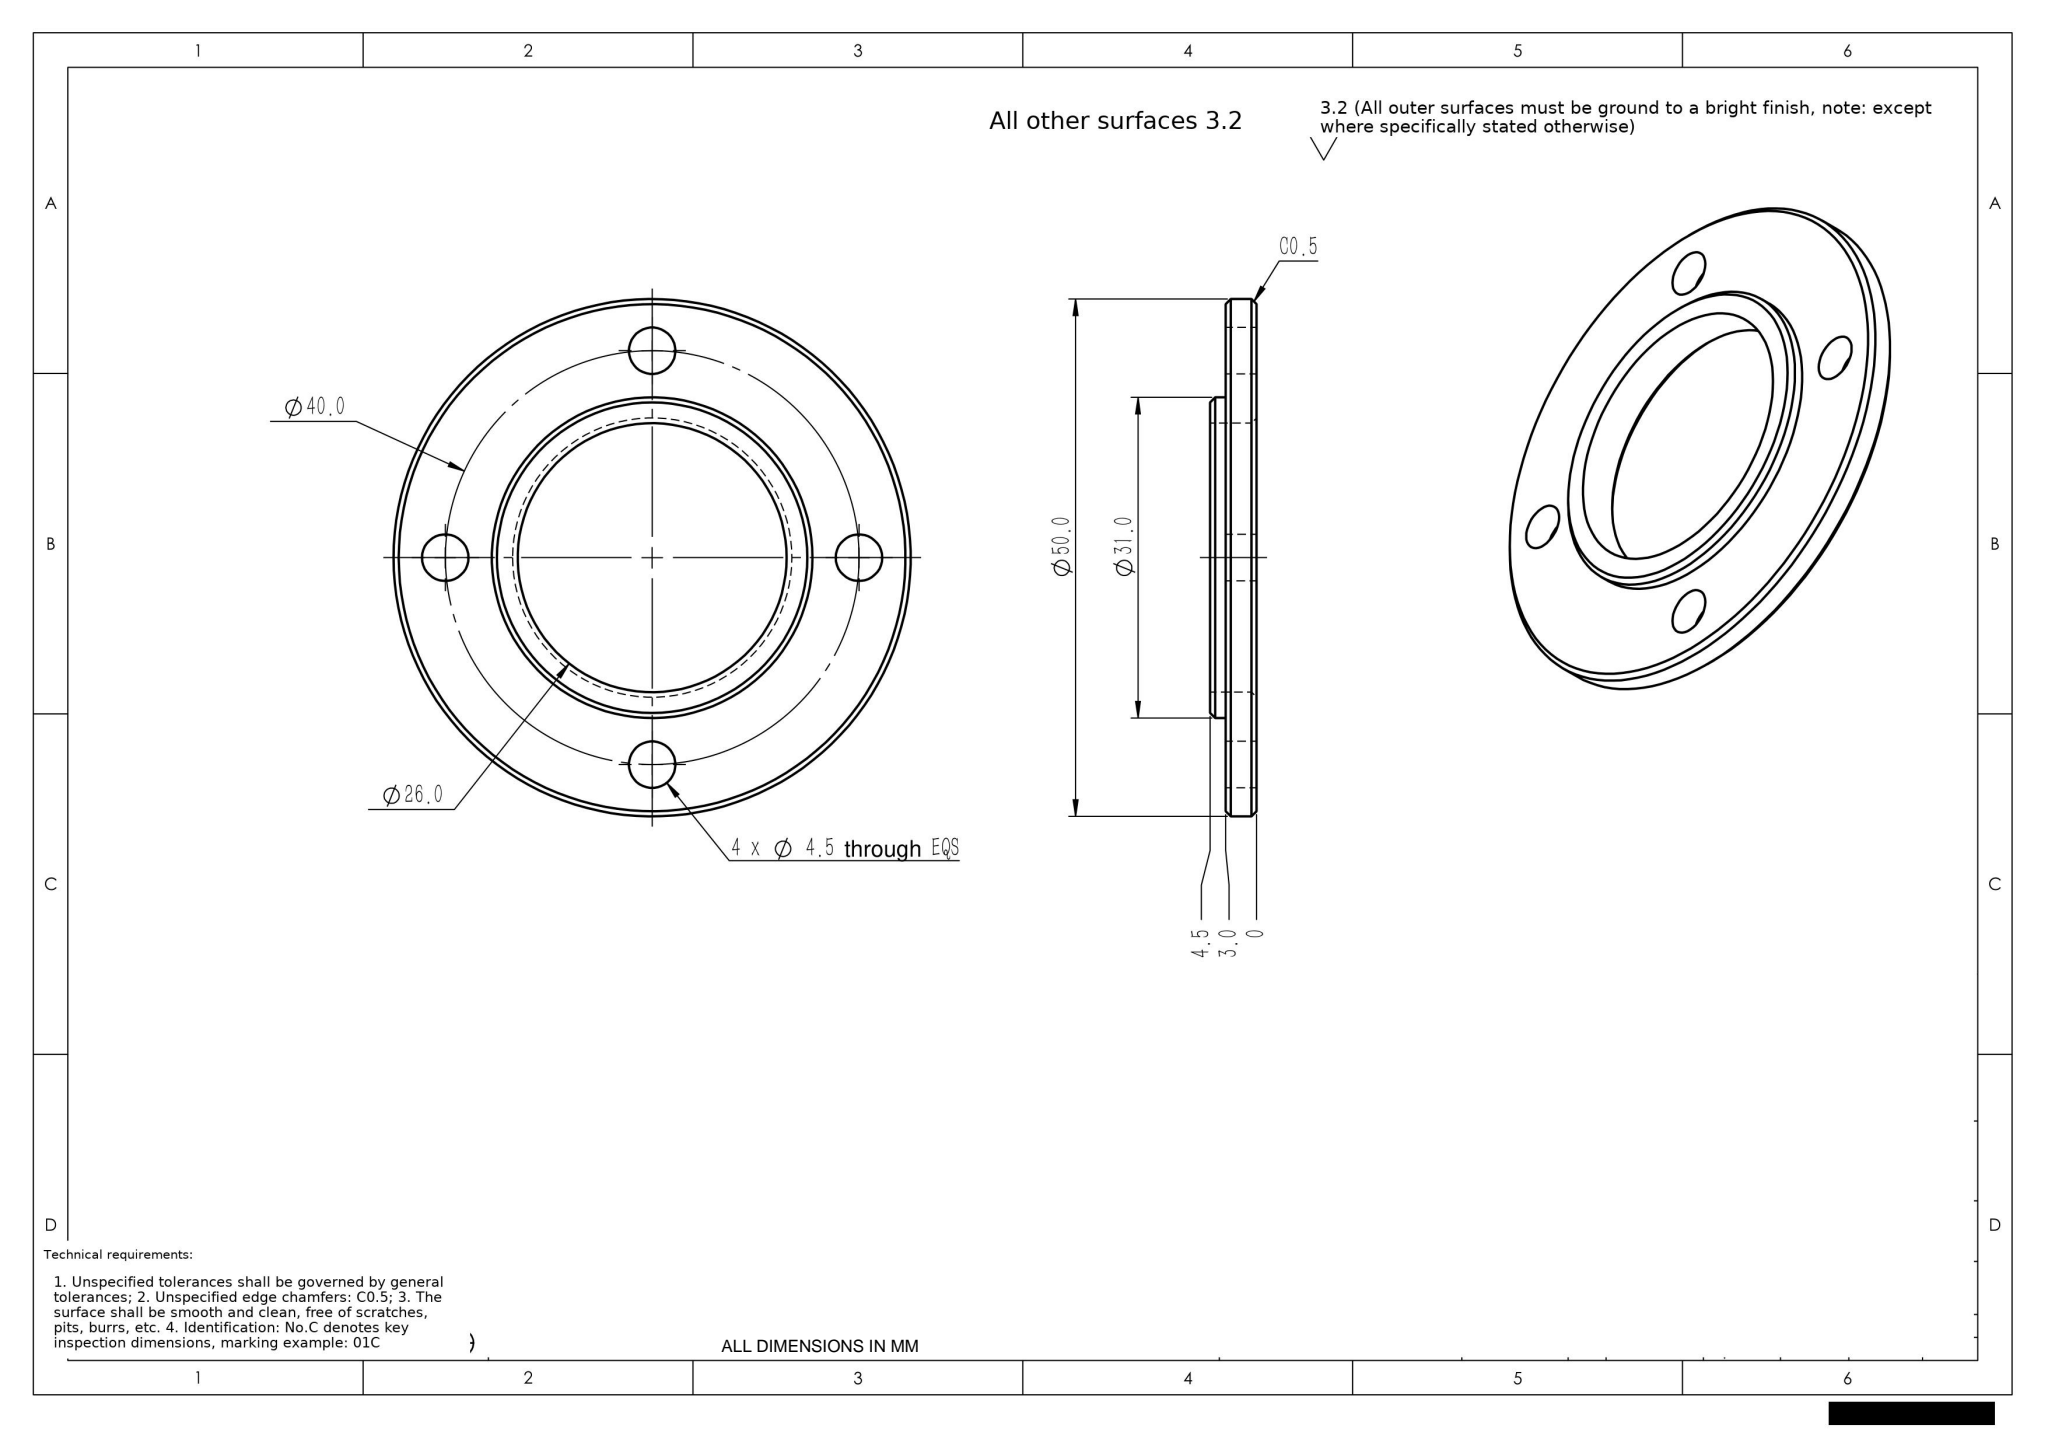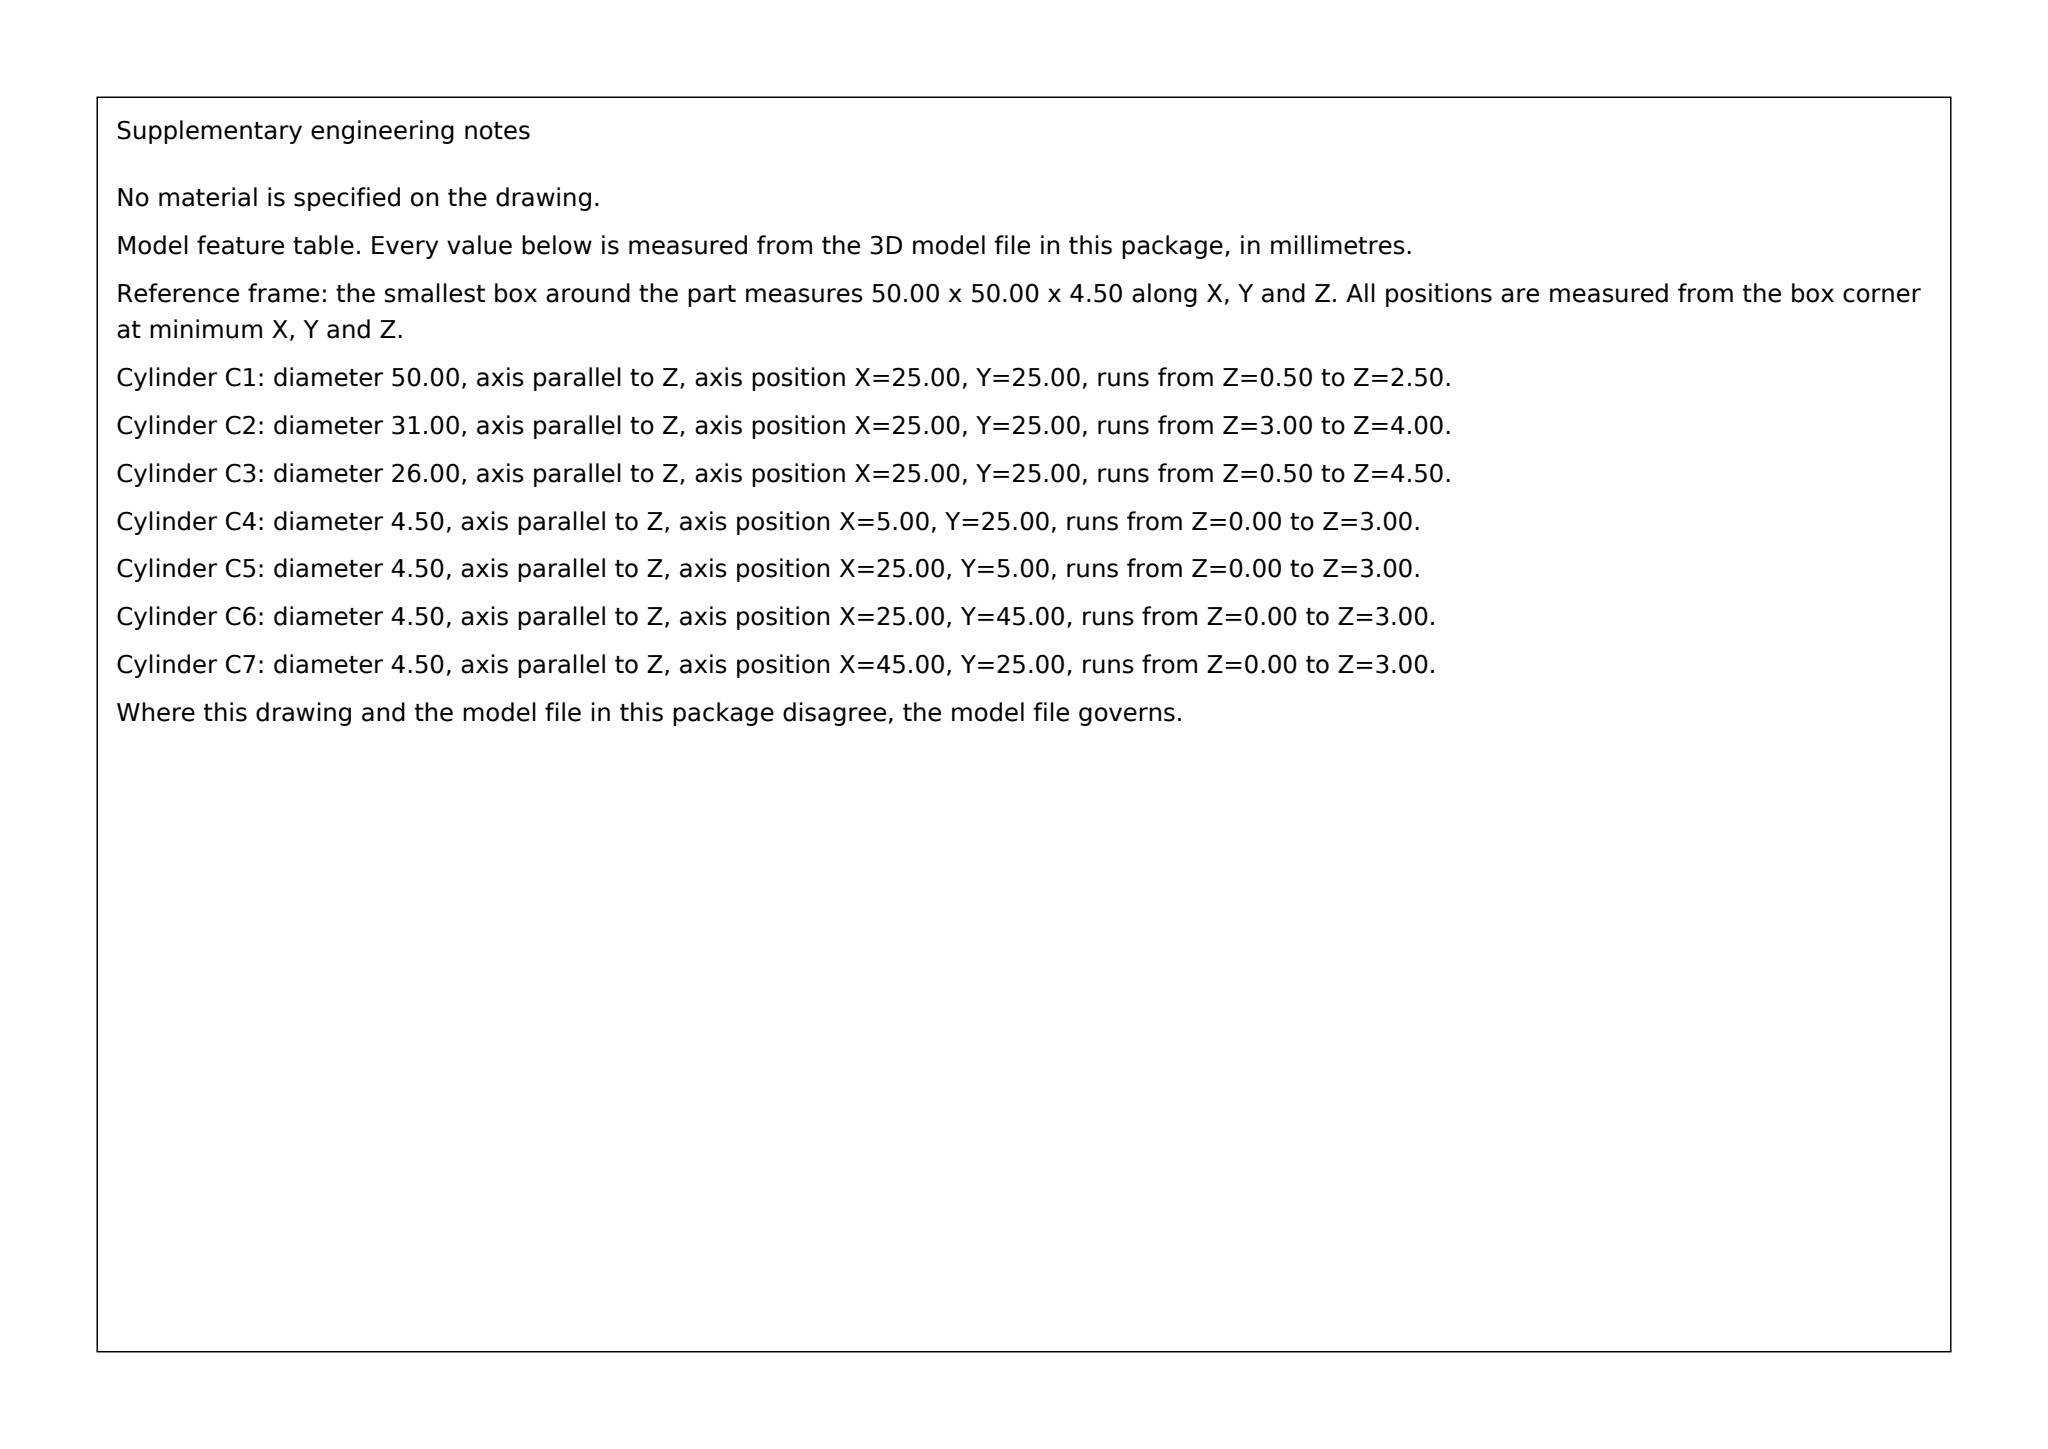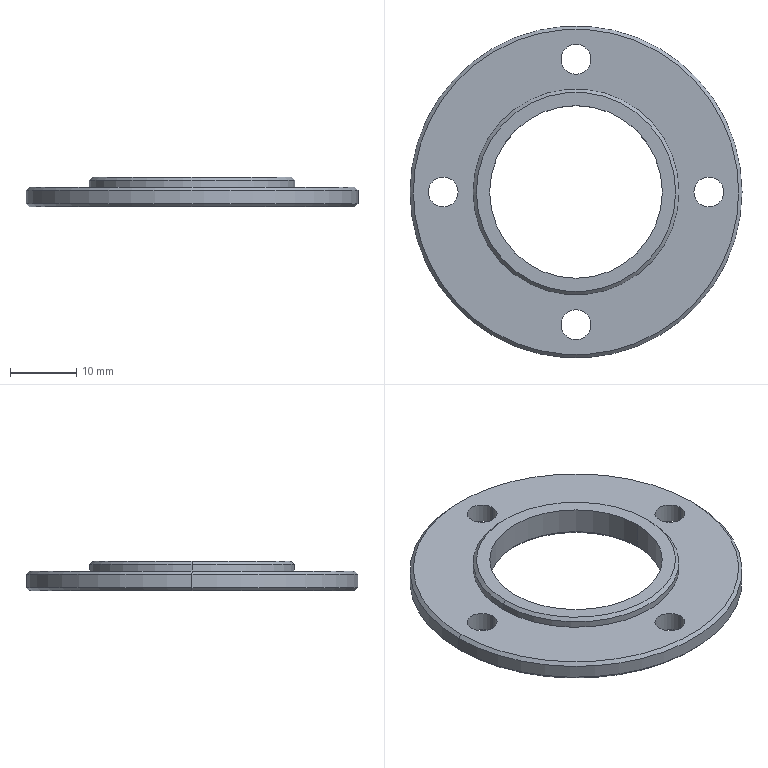Part | SolidWorks | mm | 1 solid | 25 faces | box 50 x 50 x 4.5 mm | volume 4381 mm3 | cylinder 14 | cone 8 | plane 3 | commonest cylinder face diameters 4.5 x8 26 x2 50 x2 31 x2
build123d program:
from build123d import *

# Parameters (mm, degrees)
SKETCH1_R                  = 15.5
BOSS_EXTRUDE1_DEPTH        = 1.5
SKETCH2_R                  = 25
BOSS_EXTRUDE2_DEPTH        = 3
SKETCH3_R                  = 13
CUT_EXTRUDE1_DEPTH         = 36.641
F_4_5_4_5_DIAMETER_HOLE1_D = 4.5
CHAMFER1_SIZE              = 0.5


with BuildPart() as part:
    # Sketch1 → Boss-Extrude1 (new body)
    with BuildSketch(Plane.XY):
        Circle(SKETCH1_R)
    extrude(amount=BOSS_EXTRUDE1_DEPTH)

    # Sketch2 → Boss-Extrude2 (add)
    with BuildSketch(Plane(origin=(0, 0, 0), x_dir=(-1, 0, 0), z_dir=(0, 0, -1))):
        Circle(SKETCH2_R)
    extrude(amount=BOSS_EXTRUDE2_DEPTH)

    # Sketch3 → Cut-Extrude1 (cut, through all)
    with BuildSketch(Plane.XY.offset(1.5)):
        Circle(SKETCH3_R)
    extrude(amount=-CUT_EXTRUDE1_DEPTH, mode=Mode.SUBTRACT)

    # 4.5 _4.5_ Diameter Hole1 (through all)
    with Locations(Plane(origin=(0, 0, -3), x_dir=(-1, 0, 0), z_dir=(0, 0, -1))):
        with Locations((0, -20), (0, 20), (-20, 0), (20, 0)):
            Hole(F_4_5_4_5_DIAMETER_HOLE1_D / 2)

    # Chamfer1
    chamfer1_edges = [part.edges().sort_by_distance(p)[0] for p in [
        (-13, 0, -3),
        (-15.5, 0, 1.5),
        (25, 0, 0),
        (25, 0, -3),
    ]]
    chamfer(chamfer1_edges, length=CHAMFER1_SIZE)


solid = part.part
STEP:
#1=CARTESIAN_POINT('',(15.,0.,1.5));
#2=VERTEX_POINT('',#1);
#3=CARTESIAN_POINT('',(-15.,0.,1.5));
#4=VERTEX_POINT('',#3);
#5=CARTESIAN_POINT('',(0.,0.,1.5));
#6=DIRECTION('',(0.,0.,1.));
#7=DIRECTION('',(1.,0.,0.));
#8=AXIS2_PLACEMENT_3D('',#5,#6,#7);
#9=CIRCLE('',#8,15.);
#10=EDGE_CURVE('',#2,#4,#9,.T.);
#11=ORIENTED_EDGE('',*,*,#10,.F.);
#12=CARTESIAN_POINT('',(15.5,0.,1.));
#13=VERTEX_POINT('',#12);
#14=CARTESIAN_POINT('',(15.,0.,1.5));
#15=DIRECTION('',(0.7071,0.,-0.7071));
#16=VECTOR('',#15,1000.);
#17=LINE('',#14,#16);
#18=EDGE_CURVE('',#2,#13,#17,.T.);
#19=ORIENTED_EDGE('',*,*,#18,.T.);
#20=CARTESIAN_POINT('',(-15.5,0.,1.));
#21=VERTEX_POINT('',#20);
#22=CARTESIAN_POINT('',(0.,0.,1.));
#23=DIRECTION('',(0.,0.,-1.));
#24=DIRECTION('',(1.,0.,0.));
#25=AXIS2_PLACEMENT_3D('',#22,#23,#24);
#26=CIRCLE('',#25,15.5);
#27=EDGE_CURVE('',#21,#13,#26,.T.);
#28=ORIENTED_EDGE('',*,*,#27,.F.);
#29=CARTESIAN_POINT('',(-15.,0.,1.5));
#30=DIRECTION('',(-0.7071,0.,-0.7071));
#31=VECTOR('',#30,1000.);
#32=LINE('',#29,#31);
#33=EDGE_CURVE('',#4,#21,#32,.T.);
#34=ORIENTED_EDGE('',*,*,#33,.F.);
#35=EDGE_LOOP('',(#11,#19,#28,#34));
#36=FACE_OUTER_BOUND('',#35,.T.);
#37=CARTESIAN_POINT('',(0.,0.,1.5));
#38=DIRECTION('',(0.,0.,-1.));
#39=DIRECTION('',(-1.,0.,0.));
#40=AXIS2_PLACEMENT_3D('',#37,#38,#39);
#41=CONICAL_SURFACE('',#40,15.,0.7854);
#42=ADVANCED_FACE('',(#36),#41,.T.);
#43=CARTESIAN_POINT('',(24.5,0.,0.));
#44=VERTEX_POINT('',#43);
#45=CARTESIAN_POINT('',(-24.5,0.,0.));
#46=VERTEX_POINT('',#45);
#47=CARTESIAN_POINT('',(0.,0.,0.));
#48=DIRECTION('',(0.,0.,1.));
#49=DIRECTION('',(-1.,0.,0.));
#50=AXIS2_PLACEMENT_3D('',#47,#48,#49);
#51=CIRCLE('',#50,24.5);
#52=EDGE_CURVE('',#44,#46,#51,.T.);
#53=ORIENTED_EDGE('',*,*,#52,.F.);
#54=CARTESIAN_POINT('',(25.,0.,-0.5));
#55=VERTEX_POINT('',#54);
#56=CARTESIAN_POINT('',(25.,0.,-0.5));
#57=DIRECTION('',(0.7071,0.,-0.7071));
#58=VECTOR('',#57,1000.);
#59=LINE('',#56,#58);
#60=EDGE_CURVE('',#44,#55,#59,.T.);
#61=ORIENTED_EDGE('',*,*,#60,.T.);
#62=CARTESIAN_POINT('',(-25.,0.,-0.5));
#63=VERTEX_POINT('',#62);
#64=CARTESIAN_POINT('',(0.,0.,-0.5));
#65=DIRECTION('',(0.,0.,-1.));
#66=DIRECTION('',(-1.,0.,0.));
#67=AXIS2_PLACEMENT_3D('',#64,#65,#66);
#68=CIRCLE('',#67,25.);
#69=EDGE_CURVE('',#63,#55,#68,.T.);
#70=ORIENTED_EDGE('',*,*,#69,.F.);
#71=CARTESIAN_POINT('',(-25.,0.,-0.5));
#72=DIRECTION('',(-0.7071,0.,-0.7071));
#73=VECTOR('',#72,1000.);
#74=LINE('',#71,#73);
#75=EDGE_CURVE('',#46,#63,#74,.T.);
#76=ORIENTED_EDGE('',*,*,#75,.F.);
#77=EDGE_LOOP('',(#53,#61,#70,#76));
#78=FACE_OUTER_BOUND('',#77,.T.);
#79=CARTESIAN_POINT('',(0.,0.,-0.5));
#80=DIRECTION('',(0.,0.,-1.));
#81=DIRECTION('',(-1.,0.,0.));
#82=AXIS2_PLACEMENT_3D('',#79,#80,#81);
#83=CONICAL_SURFACE('',#82,25.,0.7854);
#84=ADVANCED_FACE('',(#78),#83,.T.);
#85=CARTESIAN_POINT('',(-24.5,0.,-3.));
#86=VERTEX_POINT('',#85);
#87=CARTESIAN_POINT('',(24.5,0.,-3.));
#88=VERTEX_POINT('',#87);
#89=CARTESIAN_POINT('',(0.,0.,-3.));
#90=DIRECTION('',(0.,0.,-1.));
#91=DIRECTION('',(-1.,0.,0.));
#92=AXIS2_PLACEMENT_3D('',#89,#90,#91);
#93=CIRCLE('',#92,24.5);
#94=EDGE_CURVE('',#86,#88,#93,.T.);
#95=ORIENTED_EDGE('',*,*,#94,.F.);
#96=CARTESIAN_POINT('',(-25.,0.,-2.5));
#97=VERTEX_POINT('',#96);
#98=CARTESIAN_POINT('',(-24.5,0.,-3.));
#99=DIRECTION('',(-0.7071,0.,0.7071));
#100=VECTOR('',#99,1000.);
#101=LINE('',#98,#100);
#102=EDGE_CURVE('',#86,#97,#101,.T.);
#103=ORIENTED_EDGE('',*,*,#102,.T.);
#104=CARTESIAN_POINT('',(25.,0.,-2.5));
#105=VERTEX_POINT('',#104);
#106=CARTESIAN_POINT('',(0.,0.,-2.5));
#107=DIRECTION('',(0.,0.,1.));
#108=DIRECTION('',(-1.,0.,0.));
#109=AXIS2_PLACEMENT_3D('',#106,#107,#108);
#110=CIRCLE('',#109,25.);
#111=EDGE_CURVE('',#105,#97,#110,.T.);
#112=ORIENTED_EDGE('',*,*,#111,.F.);
#113=CARTESIAN_POINT('',(24.5,0.,-3.));
#114=DIRECTION('',(0.7071,0.,0.7071));
#115=VECTOR('',#114,1000.);
#116=LINE('',#113,#115);
#117=EDGE_CURVE('',#88,#105,#116,.T.);
#118=ORIENTED_EDGE('',*,*,#117,.F.);
#119=EDGE_LOOP('',(#95,#103,#112,#118));
#120=FACE_OUTER_BOUND('',#119,.T.);
#121=CARTESIAN_POINT('',(0.,0.,-3.));
#122=DIRECTION('',(0.,0.,1.));
#123=DIRECTION('',(1.,0.,0.));
#124=AXIS2_PLACEMENT_3D('',#121,#122,#123);
#125=CONICAL_SURFACE('',#124,24.5,0.7854);
#126=ADVANCED_FACE('',(#120),#125,.T.);
#127=CARTESIAN_POINT('',(13.,0.,-2.5));
#128=VERTEX_POINT('',#127);
#129=CARTESIAN_POINT('',(-13.,0.,-2.5));
#130=VERTEX_POINT('',#129);
#131=CARTESIAN_POINT('',(0.,0.,-2.5));
#132=DIRECTION('',(0.,0.,-1.));
#133=DIRECTION('',(-1.,0.,0.));
#134=AXIS2_PLACEMENT_3D('',#131,#132,#133);
#135=CIRCLE('',#134,13.);
#136=EDGE_CURVE('',#128,#130,#135,.T.);
#137=ORIENTED_EDGE('',*,*,#136,.F.);
#138=CARTESIAN_POINT('',(13.5,0.,-3.));
#139=VERTEX_POINT('',#138);
#140=CARTESIAN_POINT('',(13.5,0.,-3.));
#141=DIRECTION('',(0.7071,0.,-0.7071));
#142=VECTOR('',#141,1000.);
#143=LINE('',#140,#142);
#144=EDGE_CURVE('',#128,#139,#143,.T.);
#145=ORIENTED_EDGE('',*,*,#144,.T.);
#146=CARTESIAN_POINT('',(-13.5,0.,-3.));
#147=VERTEX_POINT('',#146);
#148=CARTESIAN_POINT('',(0.,0.,-3.));
#149=DIRECTION('',(0.,0.,1.));
#150=DIRECTION('',(-1.,0.,0.));
#151=AXIS2_PLACEMENT_3D('',#148,#149,#150);
#152=CIRCLE('',#151,13.5);
#153=EDGE_CURVE('',#147,#139,#152,.T.);
#154=ORIENTED_EDGE('',*,*,#153,.F.);
#155=CARTESIAN_POINT('',(-13.5,0.,-3.));
#156=DIRECTION('',(-0.7071,0.,-0.7071));
#157=VECTOR('',#156,1000.);
#158=LINE('',#155,#157);
#159=EDGE_CURVE('',#130,#147,#158,.T.);
#160=ORIENTED_EDGE('',*,*,#159,.F.);
#161=EDGE_LOOP('',(#137,#145,#154,#160));
#162=FACE_OUTER_BOUND('',#161,.T.);
#163=CARTESIAN_POINT('',(0.,0.,-3.));
#164=DIRECTION('',(0.,0.,-1.));
#165=DIRECTION('',(-1.,0.,0.));
#166=AXIS2_PLACEMENT_3D('',#163,#164,#165);
#167=CONICAL_SURFACE('',#166,13.5,0.7854);
#168=ADVANCED_FACE('',(#162),#167,.F.);
#169=CARTESIAN_POINT('',(2.25,-20.,0.));
#170=VERTEX_POINT('',#169);
#171=CARTESIAN_POINT('',(-2.25,-20.,0.));
#172=VERTEX_POINT('',#171);
#173=CARTESIAN_POINT('',(0.,-20.,0.));
#174=DIRECTION('',(0.,0.,-1.));
#175=DIRECTION('',(-1.,0.,0.));
#176=AXIS2_PLACEMENT_3D('',#173,#174,#175);
#177=CIRCLE('',#176,2.25);
#178=EDGE_CURVE('',#170,#172,#177,.T.);
#179=ORIENTED_EDGE('',*,*,#178,.F.);
#180=CARTESIAN_POINT('',(2.25,-20.,-3.));
#181=VERTEX_POINT('',#180);
#182=CARTESIAN_POINT('',(2.25,-20.,-3.));
#183=DIRECTION('',(0.,0.,-1.));
#184=VECTOR('',#183,1000.);
#185=LINE('',#182,#184);
#186=EDGE_CURVE('',#170,#181,#185,.T.);
#187=ORIENTED_EDGE('',*,*,#186,.T.);
#188=CARTESIAN_POINT('',(-2.25,-20.,-3.));
#189=VERTEX_POINT('',#188);
#190=CARTESIAN_POINT('',(0.,-20.,-3.));
#191=DIRECTION('',(0.,0.,-1.));
#192=DIRECTION('',(-1.,0.,0.));
#193=AXIS2_PLACEMENT_3D('',#190,#191,#192);
#194=CIRCLE('',#193,2.25);
#195=EDGE_CURVE('',#181,#189,#194,.T.);
#196=ORIENTED_EDGE('',*,*,#195,.T.);
#197=CARTESIAN_POINT('',(-2.25,-20.,-3.));
#198=DIRECTION('',(0.,0.,-1.));
#199=VECTOR('',#198,1000.);
#200=LINE('',#197,#199);
#201=EDGE_CURVE('',#172,#189,#200,.T.);
#202=ORIENTED_EDGE('',*,*,#201,.F.);
#203=EDGE_LOOP('',(#179,#187,#196,#202));
#204=FACE_OUTER_BOUND('',#203,.T.);
#205=CARTESIAN_POINT('',(0.,-20.,-3.));
#206=DIRECTION('',(0.,0.,-1.));
#207=DIRECTION('',(-1.,0.,0.));
#208=AXIS2_PLACEMENT_3D('',#205,#206,#207);
#209=CYLINDRICAL_SURFACE('',#208,2.25);
#210=ADVANCED_FACE('',(#204),#209,.F.);
#211=CARTESIAN_POINT('',(2.25,20.,0.));
#212=VERTEX_POINT('',#211);
#213=CARTESIAN_POINT('',(-2.25,20.,0.));
#214=VERTEX_POINT('',#213);
#215=CARTESIAN_POINT('',(0.,20.,0.));
#216=DIRECTION('',(0.,0.,-1.));
#217=DIRECTION('',(-1.,0.,0.));
#218=AXIS2_PLACEMENT_3D('',#215,#216,#217);
#219=CIRCLE('',#218,2.25);
#220=EDGE_CURVE('',#212,#214,#219,.T.);
#221=ORIENTED_EDGE('',*,*,#220,.F.);
#222=CARTESIAN_POINT('',(2.25,20.,-3.));
#223=VERTEX_POINT('',#222);
#224=CARTESIAN_POINT('',(2.25,20.,-3.));
#225=DIRECTION('',(0.,0.,-1.));
#226=VECTOR('',#225,1000.);
#227=LINE('',#224,#226);
#228=EDGE_CURVE('',#212,#223,#227,.T.);
#229=ORIENTED_EDGE('',*,*,#228,.T.);
#230=CARTESIAN_POINT('',(-2.25,20.,-3.));
#231=VERTEX_POINT('',#230);
#232=CARTESIAN_POINT('',(0.,20.,-3.));
#233=DIRECTION('',(0.,0.,-1.));
#234=DIRECTION('',(-1.,0.,0.));
#235=AXIS2_PLACEMENT_3D('',#232,#233,#234);
#236=CIRCLE('',#235,2.25);
#237=EDGE_CURVE('',#223,#231,#236,.T.);
#238=ORIENTED_EDGE('',*,*,#237,.T.);
#239=CARTESIAN_POINT('',(-2.25,20.,-3.));
#240=DIRECTION('',(0.,0.,-1.));
#241=VECTOR('',#240,1000.);
#242=LINE('',#239,#241);
#243=EDGE_CURVE('',#214,#231,#242,.T.);
#244=ORIENTED_EDGE('',*,*,#243,.F.);
#245=EDGE_LOOP('',(#221,#229,#238,#244));
#246=FACE_OUTER_BOUND('',#245,.T.);
#247=CARTESIAN_POINT('',(0.,20.,-3.));
#248=DIRECTION('',(0.,0.,-1.));
#249=DIRECTION('',(-1.,0.,0.));
#250=AXIS2_PLACEMENT_3D('',#247,#248,#249);
#251=CYLINDRICAL_SURFACE('',#250,2.25);
#252=ADVANCED_FACE('',(#246),#251,.F.);
#253=CARTESIAN_POINT('',(22.25,0.,0.));
#254=VERTEX_POINT('',#253);
#255=CARTESIAN_POINT('',(17.75,0.,0.));
#256=VERTEX_POINT('',#255);
#257=CARTESIAN_POINT('',(20.,0.,0.));
#258=DIRECTION('',(0.,0.,-1.));
#259=DIRECTION('',(-1.,0.,0.));
#260=AXIS2_PLACEMENT_3D('',#257,#258,#259);
#261=CIRCLE('',#260,2.25);
#262=EDGE_CURVE('',#254,#256,#261,.T.);
#263=ORIENTED_EDGE('',*,*,#262,.F.);
#264=CARTESIAN_POINT('',(22.25,0.,-3.));
#265=VERTEX_POINT('',#264);
#266=CARTESIAN_POINT('',(22.25,0.,-3.));
#267=DIRECTION('',(0.,0.,-1.));
#268=VECTOR('',#267,1000.);
#269=LINE('',#266,#268);
#270=EDGE_CURVE('',#254,#265,#269,.T.);
#271=ORIENTED_EDGE('',*,*,#270,.T.);
#272=CARTESIAN_POINT('',(17.75,0.,-3.));
#273=VERTEX_POINT('',#272);
#274=CARTESIAN_POINT('',(20.,0.,-3.));
#275=DIRECTION('',(0.,0.,-1.));
#276=DIRECTION('',(-1.,0.,0.));
#277=AXIS2_PLACEMENT_3D('',#274,#275,#276);
#278=CIRCLE('',#277,2.25);
#279=EDGE_CURVE('',#265,#273,#278,.T.);
#280=ORIENTED_EDGE('',*,*,#279,.T.);
#281=CARTESIAN_POINT('',(17.75,0.,-3.));
#282=DIRECTION('',(0.,0.,-1.));
#283=VECTOR('',#282,1000.);
#284=LINE('',#281,#283);
#285=EDGE_CURVE('',#256,#273,#284,.T.);
#286=ORIENTED_EDGE('',*,*,#285,.F.);
#287=EDGE_LOOP('',(#263,#271,#280,#286));
#288=FACE_OUTER_BOUND('',#287,.T.);
#289=CARTESIAN_POINT('',(20.,0.,-3.));
#290=DIRECTION('',(0.,0.,-1.));
#291=DIRECTION('',(-1.,0.,0.));
#292=AXIS2_PLACEMENT_3D('',#289,#290,#291);
#293=CYLINDRICAL_SURFACE('',#292,2.25);
#294=ADVANCED_FACE('',(#288),#293,.F.);
#295=CARTESIAN_POINT('',(-17.75,0.,0.));
#296=VERTEX_POINT('',#295);
#297=CARTESIAN_POINT('',(-22.25,0.,0.));
#298=VERTEX_POINT('',#297);
#299=CARTESIAN_POINT('',(-20.,0.,0.));
#300=DIRECTION('',(0.,0.,-1.));
#301=DIRECTION('',(-1.,0.,0.));
#302=AXIS2_PLACEMENT_3D('',#299,#300,#301);
#303=CIRCLE('',#302,2.25);
#304=EDGE_CURVE('',#296,#298,#303,.T.);
#305=ORIENTED_EDGE('',*,*,#304,.F.);
#306=CARTESIAN_POINT('',(-17.75,0.,-3.));
#307=VERTEX_POINT('',#306);
#308=CARTESIAN_POINT('',(-17.75,0.,-3.));
#309=DIRECTION('',(0.,0.,-1.));
#310=VECTOR('',#309,1000.);
#311=LINE('',#308,#310);
#312=EDGE_CURVE('',#296,#307,#311,.T.);
#313=ORIENTED_EDGE('',*,*,#312,.T.);
#314=CARTESIAN_POINT('',(-22.25,0.,-3.));
#315=VERTEX_POINT('',#314);
#316=CARTESIAN_POINT('',(-20.,0.,-3.));
#317=DIRECTION('',(0.,0.,-1.));
#318=DIRECTION('',(-1.,0.,0.));
#319=AXIS2_PLACEMENT_3D('',#316,#317,#318);
#320=CIRCLE('',#319,2.25);
#321=EDGE_CURVE('',#307,#315,#320,.T.);
#322=ORIENTED_EDGE('',*,*,#321,.T.);
#323=CARTESIAN_POINT('',(-22.25,0.,-3.));
#324=DIRECTION('',(0.,0.,-1.));
#325=VECTOR('',#324,1000.);
#326=LINE('',#323,#325);
#327=EDGE_CURVE('',#298,#315,#326,.T.);
#328=ORIENTED_EDGE('',*,*,#327,.F.);
#329=EDGE_LOOP('',(#305,#313,#322,#328));
#330=FACE_OUTER_BOUND('',#329,.T.);
#331=CARTESIAN_POINT('',(-20.,0.,-3.));
#332=DIRECTION('',(0.,0.,-1.));
#333=DIRECTION('',(-1.,0.,0.));
#334=AXIS2_PLACEMENT_3D('',#331,#332,#333);
#335=CYLINDRICAL_SURFACE('',#334,2.25);
#336=ADVANCED_FACE('',(#330),#335,.F.);
#337=ORIENTED_EDGE('',*,*,#136,.T.);
#338=CARTESIAN_POINT('',(-13.,0.,1.5));
#339=VERTEX_POINT('',#338);
#340=CARTESIAN_POINT('',(-13.,0.,-3.));
#341=DIRECTION('',(0.,0.,1.));
#342=VECTOR('',#341,1000.);
#343=LINE('',#340,#342);
#344=EDGE_CURVE('',#130,#339,#343,.T.);
#345=ORIENTED_EDGE('',*,*,#344,.T.);
#346=CARTESIAN_POINT('',(13.,0.,1.5));
#347=VERTEX_POINT('',#346);
#348=CARTESIAN_POINT('',(0.,0.,1.5));
#349=DIRECTION('',(0.,0.,1.));
#350=DIRECTION('',(1.,0.,0.));
#351=AXIS2_PLACEMENT_3D('',#348,#349,#350);
#352=CIRCLE('',#351,13.);
#353=EDGE_CURVE('',#339,#347,#352,.T.);
#354=ORIENTED_EDGE('',*,*,#353,.T.);
#355=CARTESIAN_POINT('',(13.,0.,-3.));
#356=DIRECTION('',(0.,0.,1.));
#357=VECTOR('',#356,1000.);
#358=LINE('',#355,#357);
#359=EDGE_CURVE('',#128,#347,#358,.T.);
#360=ORIENTED_EDGE('',*,*,#359,.F.);
#361=EDGE_LOOP('',(#337,#345,#354,#360));
#362=FACE_OUTER_BOUND('',#361,.T.);
#363=CARTESIAN_POINT('',(0.,0.,-3.));
#364=DIRECTION('',(0.,0.,1.));
#365=DIRECTION('',(1.,0.,0.));
#366=AXIS2_PLACEMENT_3D('',#363,#364,#365);
#367=CYLINDRICAL_SURFACE('',#366,13.);
#368=ADVANCED_FACE('',(#362),#367,.F.);
#369=ORIENTED_EDGE('',*,*,#111,.T.);
#370=CARTESIAN_POINT('',(-25.,0.,-3.));
#371=DIRECTION('',(0.,0.,1.));
#372=VECTOR('',#371,1000.);
#373=LINE('',#370,#372);
#374=EDGE_CURVE('',#97,#63,#373,.T.);
#375=ORIENTED_EDGE('',*,*,#374,.T.);
#376=ORIENTED_EDGE('',*,*,#69,.T.);
#377=CARTESIAN_POINT('',(25.,0.,-3.));
#378=DIRECTION('',(0.,0.,1.));
#379=VECTOR('',#378,1000.);
#380=LINE('',#377,#379);
#381=EDGE_CURVE('',#105,#55,#380,.T.);
#382=ORIENTED_EDGE('',*,*,#381,.F.);
#383=EDGE_LOOP('',(#369,#375,#376,#382));
#384=FACE_OUTER_BOUND('',#383,.T.);
#385=CARTESIAN_POINT('',(0.,0.,-3.));
#386=DIRECTION('',(0.,0.,1.));
#387=DIRECTION('',(1.,0.,0.));
#388=AXIS2_PLACEMENT_3D('',#385,#386,#387);
#389=CYLINDRICAL_SURFACE('',#388,25.);
#390=ADVANCED_FACE('',(#384),#389,.T.);
#391=ORIENTED_EDGE('',*,*,#27,.T.);
#392=CARTESIAN_POINT('',(15.5,0.,0.));
#393=VERTEX_POINT('',#392);
#394=CARTESIAN_POINT('',(15.5,0.,1.5));
#395=DIRECTION('',(0.,0.,-1.));
#396=VECTOR('',#395,1000.);
#397=LINE('',#394,#396);
#398=EDGE_CURVE('',#13,#393,#397,.T.);
#399=ORIENTED_EDGE('',*,*,#398,.T.);
#400=CARTESIAN_POINT('',(-15.5,0.,0.));
#401=VERTEX_POINT('',#400);
#402=CARTESIAN_POINT('',(0.,0.,0.));
#403=DIRECTION('',(0.,0.,-1.));
#404=DIRECTION('',(-1.,0.,0.));
#405=AXIS2_PLACEMENT_3D('',#402,#403,#404);
#406=CIRCLE('',#405,15.5);
#407=EDGE_CURVE('',#401,#393,#406,.T.);
#408=ORIENTED_EDGE('',*,*,#407,.F.);
#409=CARTESIAN_POINT('',(-15.5,0.,1.5));
#410=DIRECTION('',(0.,0.,-1.));
#411=VECTOR('',#410,1000.);
#412=LINE('',#409,#411);
#413=EDGE_CURVE('',#21,#401,#412,.T.);
#414=ORIENTED_EDGE('',*,*,#413,.F.);
#415=EDGE_LOOP('',(#391,#399,#408,#414));
#416=FACE_OUTER_BOUND('',#415,.T.);
#417=CARTESIAN_POINT('',(0.,0.,1.5));
#418=DIRECTION('',(0.,0.,-1.));
#419=DIRECTION('',(-1.,0.,0.));
#420=AXIS2_PLACEMENT_3D('',#417,#418,#419);
#421=CYLINDRICAL_SURFACE('',#420,15.5);
#422=ADVANCED_FACE('',(#416),#421,.T.);
#423=ORIENTED_EDGE('',*,*,#398,.F.);
#424=CARTESIAN_POINT('',(0.,0.,1.));
#425=DIRECTION('',(0.,0.,-1.));
#426=DIRECTION('',(1.,0.,0.));
#427=AXIS2_PLACEMENT_3D('',#424,#425,#426);
#428=CIRCLE('',#427,15.5);
#429=EDGE_CURVE('',#13,#21,#428,.T.);
#430=ORIENTED_EDGE('',*,*,#429,.T.);
#431=ORIENTED_EDGE('',*,*,#413,.T.);
#432=CARTESIAN_POINT('',(0.,0.,0.));
#433=DIRECTION('',(0.,0.,-1.));
#434=DIRECTION('',(-1.,0.,0.));
#435=AXIS2_PLACEMENT_3D('',#432,#433,#434);
#436=CIRCLE('',#435,15.5);
#437=EDGE_CURVE('',#393,#401,#436,.T.);
#438=ORIENTED_EDGE('',*,*,#437,.F.);
#439=EDGE_LOOP('',(#423,#430,#431,#438));
#440=FACE_OUTER_BOUND('',#439,.T.);
#441=CARTESIAN_POINT('',(0.,0.,1.5));
#442=DIRECTION('',(0.,0.,-1.));
#443=DIRECTION('',(-1.,0.,0.));
#444=AXIS2_PLACEMENT_3D('',#441,#442,#443);
#445=CYLINDRICAL_SURFACE('',#444,15.5);
#446=ADVANCED_FACE('',(#440),#445,.T.);
#447=CARTESIAN_POINT('',(0.,0.,1.5));
#448=DIRECTION('',(0.,0.,1.));
#449=DIRECTION('',(1.,0.,0.));
#450=AXIS2_PLACEMENT_3D('',#447,#448,#449);
#451=CIRCLE('',#450,15.);
#452=EDGE_CURVE('',#4,#2,#451,.T.);
#453=ORIENTED_EDGE('',*,*,#452,.T.);
#454=ORIENTED_EDGE('',*,*,#10,.T.);
#455=EDGE_LOOP('',(#453,#454));
#456=FACE_OUTER_BOUND('',#455,.T.);
#457=CARTESIAN_POINT('',(0.,0.,1.5));
#458=DIRECTION('',(0.,0.,1.));
#459=DIRECTION('',(1.,0.,0.));
#460=AXIS2_PLACEMENT_3D('',#457,#458,#459);
#461=CIRCLE('',#460,13.);
#462=EDGE_CURVE('',#347,#339,#461,.T.);
#463=ORIENTED_EDGE('',*,*,#462,.F.);
#464=ORIENTED_EDGE('',*,*,#353,.F.);
#465=EDGE_LOOP('',(#463,#464));
#466=FACE_BOUND('',#465,.T.);
#467=CARTESIAN_POINT('',(0.,0.,1.5));
#468=DIRECTION('',(0.,0.,1.));
#469=DIRECTION('',(1.,0.,0.));
#470=AXIS2_PLACEMENT_3D('',#467,#468,#469);
#471=PLANE('',#470);
#472=ADVANCED_FACE('',(#456,#466),#471,.T.);
#473=ORIENTED_EDGE('',*,*,#374,.F.);
#474=CARTESIAN_POINT('',(0.,0.,-2.5));
#475=DIRECTION('',(0.,0.,1.));
#476=DIRECTION('',(-1.,0.,0.));
#477=AXIS2_PLACEMENT_3D('',#474,#475,#476);
#478=CIRCLE('',#477,25.);
#479=EDGE_CURVE('',#97,#105,#478,.T.);
#480=ORIENTED_EDGE('',*,*,#479,.T.);
#481=ORIENTED_EDGE('',*,*,#381,.T.);
#482=CARTESIAN_POINT('',(0.,0.,-0.5));
#483=DIRECTION('',(0.,0.,-1.));
#484=DIRECTION('',(-1.,0.,0.));
#485=AXIS2_PLACEMENT_3D('',#482,#483,#484);
#486=CIRCLE('',#485,25.);
#487=EDGE_CURVE('',#55,#63,#486,.T.);
#488=ORIENTED_EDGE('',*,*,#487,.T.);
#489=EDGE_LOOP('',(#473,#480,#481,#488));
#490=FACE_OUTER_BOUND('',#489,.T.);
#491=CARTESIAN_POINT('',(0.,0.,-3.));
#492=DIRECTION('',(0.,0.,1.));
#493=DIRECTION('',(1.,0.,0.));
#494=AXIS2_PLACEMENT_3D('',#491,#492,#493);
#495=CYLINDRICAL_SURFACE('',#494,25.);
#496=ADVANCED_FACE('',(#490),#495,.T.);
#497=ORIENTED_EDGE('',*,*,#153,.T.);
#498=CARTESIAN_POINT('',(0.,0.,-3.));
#499=DIRECTION('',(0.,0.,1.));
#500=DIRECTION('',(-1.,0.,0.));
#501=AXIS2_PLACEMENT_3D('',#498,#499,#500);
#502=CIRCLE('',#501,13.5);
#503=EDGE_CURVE('',#139,#147,#502,.T.);
#504=ORIENTED_EDGE('',*,*,#503,.T.);
#505=EDGE_LOOP('',(#497,#504));
#506=FACE_BOUND('',#505,.T.);
#507=CARTESIAN_POINT('',(0.,0.,-3.));
#508=DIRECTION('',(0.,0.,-1.));
#509=DIRECTION('',(-1.,0.,0.));
#510=AXIS2_PLACEMENT_3D('',#507,#508,#509);
#511=CIRCLE('',#510,24.5);
#512=EDGE_CURVE('',#88,#86,#511,.T.);
#513=ORIENTED_EDGE('',*,*,#512,.T.);
#514=ORIENTED_EDGE('',*,*,#94,.T.);
#515=EDGE_LOOP('',(#513,#514));
#516=FACE_OUTER_BOUND('',#515,.T.);
#517=CARTESIAN_POINT('',(0.,-20.,-3.));
#518=DIRECTION('',(0.,0.,-1.));
#519=DIRECTION('',(-1.,0.,0.));
#520=AXIS2_PLACEMENT_3D('',#517,#518,#519);
#521=CIRCLE('',#520,2.25);
#522=EDGE_CURVE('',#189,#181,#521,.T.);
#523=ORIENTED_EDGE('',*,*,#522,.F.);
#524=ORIENTED_EDGE('',*,*,#195,.F.);
#525=EDGE_LOOP('',(#523,#524));
#526=FACE_BOUND('',#525,.T.);
#527=CARTESIAN_POINT('',(0.,20.,-3.));
#528=DIRECTION('',(0.,0.,-1.));
#529=DIRECTION('',(-1.,0.,0.));
#530=AXIS2_PLACEMENT_3D('',#527,#528,#529);
#531=CIRCLE('',#530,2.25);
#532=EDGE_CURVE('',#231,#223,#531,.T.);
#533=ORIENTED_EDGE('',*,*,#532,.F.);
#534=ORIENTED_EDGE('',*,*,#237,.F.);
#535=EDGE_LOOP('',(#533,#534));
#536=FACE_BOUND('',#535,.T.);
#537=CARTESIAN_POINT('',(20.,0.,-3.));
#538=DIRECTION('',(0.,0.,-1.));
#539=DIRECTION('',(-1.,0.,0.));
#540=AXIS2_PLACEMENT_3D('',#537,#538,#539);
#541=CIRCLE('',#540,2.25);
#542=EDGE_CURVE('',#273,#265,#541,.T.);
#543=ORIENTED_EDGE('',*,*,#542,.F.);
#544=ORIENTED_EDGE('',*,*,#279,.F.);
#545=EDGE_LOOP('',(#543,#544));
#546=FACE_BOUND('',#545,.T.);
#547=CARTESIAN_POINT('',(-20.,0.,-3.));
#548=DIRECTION('',(0.,0.,-1.));
#549=DIRECTION('',(-1.,0.,0.));
#550=AXIS2_PLACEMENT_3D('',#547,#548,#549);
#551=CIRCLE('',#550,2.25);
#552=EDGE_CURVE('',#315,#307,#551,.T.);
#553=ORIENTED_EDGE('',*,*,#552,.F.);
#554=ORIENTED_EDGE('',*,*,#321,.F.);
#555=EDGE_LOOP('',(#553,#554));
#556=FACE_BOUND('',#555,.T.);
#557=CARTESIAN_POINT('',(0.,0.,-3.));
#558=DIRECTION('',(0.,0.,-1.));
#559=DIRECTION('',(-1.,0.,0.));
#560=AXIS2_PLACEMENT_3D('',#557,#558,#559);
#561=PLANE('',#560);
#562=ADVANCED_FACE('',(#506,#516,#526,#536,#546,#556),#561,.T.);
#563=CARTESIAN_POINT('',(0.,0.,0.));
#564=DIRECTION('',(0.,0.,1.));
#565=DIRECTION('',(-1.,0.,0.));
#566=AXIS2_PLACEMENT_3D('',#563,#564,#565);
#567=CIRCLE('',#566,24.5);
#568=EDGE_CURVE('',#46,#44,#567,.T.);
#569=ORIENTED_EDGE('',*,*,#568,.T.);
#570=ORIENTED_EDGE('',*,*,#52,.T.);
#571=EDGE_LOOP('',(#569,#570));
#572=FACE_OUTER_BOUND('',#571,.T.);
#573=CARTESIAN_POINT('',(0.,-20.,0.));
#574=DIRECTION('',(0.,0.,-1.));
#575=DIRECTION('',(-1.,0.,0.));
#576=AXIS2_PLACEMENT_3D('',#573,#574,#575);
#577=CIRCLE('',#576,2.25);
#578=EDGE_CURVE('',#172,#170,#577,.T.);
#579=ORIENTED_EDGE('',*,*,#578,.T.);
#580=ORIENTED_EDGE('',*,*,#178,.T.);
#581=EDGE_LOOP('',(#579,#580));
#582=FACE_BOUND('',#581,.T.);
#583=CARTESIAN_POINT('',(0.,20.,0.));
#584=DIRECTION('',(0.,0.,-1.));
#585=DIRECTION('',(-1.,0.,0.));
#586=AXIS2_PLACEMENT_3D('',#583,#584,#585);
#587=CIRCLE('',#586,2.25);
#588=EDGE_CURVE('',#214,#212,#587,.T.);
#589=ORIENTED_EDGE('',*,*,#588,.T.);
#590=ORIENTED_EDGE('',*,*,#220,.T.);
#591=EDGE_LOOP('',(#589,#590));
#592=FACE_BOUND('',#591,.T.);
#593=CARTESIAN_POINT('',(20.,0.,0.));
#594=DIRECTION('',(0.,0.,-1.));
#595=DIRECTION('',(-1.,0.,0.));
#596=AXIS2_PLACEMENT_3D('',#593,#594,#595);
#597=CIRCLE('',#596,2.25);
#598=EDGE_CURVE('',#256,#254,#597,.T.);
#599=ORIENTED_EDGE('',*,*,#598,.T.);
#600=ORIENTED_EDGE('',*,*,#262,.T.);
#601=EDGE_LOOP('',(#599,#600));
#602=FACE_BOUND('',#601,.T.);
#603=CARTESIAN_POINT('',(-20.,0.,0.));
#604=DIRECTION('',(0.,0.,-1.));
#605=DIRECTION('',(-1.,0.,0.));
#606=AXIS2_PLACEMENT_3D('',#603,#604,#605);
#607=CIRCLE('',#606,2.25);
#608=EDGE_CURVE('',#298,#296,#607,.T.);
#609=ORIENTED_EDGE('',*,*,#608,.T.);
#610=ORIENTED_EDGE('',*,*,#304,.T.);
#611=EDGE_LOOP('',(#609,#610));
#612=FACE_BOUND('',#611,.T.);
#613=ORIENTED_EDGE('',*,*,#407,.T.);
#614=ORIENTED_EDGE('',*,*,#437,.T.);
#615=EDGE_LOOP('',(#613,#614));
#616=FACE_BOUND('',#615,.T.);
#617=CARTESIAN_POINT('',(0.,0.,0.));
#618=DIRECTION('',(0.,0.,-1.));
#619=DIRECTION('',(-1.,0.,0.));
#620=AXIS2_PLACEMENT_3D('',#617,#618,#619);
#621=PLANE('',#620);
#622=ADVANCED_FACE('',(#572,#582,#592,#602,#612,#616),#621,.F.);
#623=ORIENTED_EDGE('',*,*,#344,.F.);
#624=CARTESIAN_POINT('',(0.,0.,-2.5));
#625=DIRECTION('',(0.,0.,-1.));
#626=DIRECTION('',(-1.,0.,0.));
#627=AXIS2_PLACEMENT_3D('',#624,#625,#626);
#628=CIRCLE('',#627,13.);
#629=EDGE_CURVE('',#130,#128,#628,.T.);
#630=ORIENTED_EDGE('',*,*,#629,.T.);
#631=ORIENTED_EDGE('',*,*,#359,.T.);
#632=ORIENTED_EDGE('',*,*,#462,.T.);
#633=EDGE_LOOP('',(#623,#630,#631,#632));
#634=FACE_OUTER_BOUND('',#633,.T.);
#635=CARTESIAN_POINT('',(0.,0.,-3.));
#636=DIRECTION('',(0.,0.,1.));
#637=DIRECTION('',(1.,0.,0.));
#638=AXIS2_PLACEMENT_3D('',#635,#636,#637);
#639=CYLINDRICAL_SURFACE('',#638,13.);
#640=ADVANCED_FACE('',(#634),#639,.F.);
#641=ORIENTED_EDGE('',*,*,#312,.F.);
#642=ORIENTED_EDGE('',*,*,#608,.F.);
#643=ORIENTED_EDGE('',*,*,#327,.T.);
#644=ORIENTED_EDGE('',*,*,#552,.T.);
#645=EDGE_LOOP('',(#641,#642,#643,#644));
#646=FACE_OUTER_BOUND('',#645,.T.);
#647=CARTESIAN_POINT('',(-20.,0.,-3.));
#648=DIRECTION('',(0.,0.,-1.));
#649=DIRECTION('',(-1.,0.,0.));
#650=AXIS2_PLACEMENT_3D('',#647,#648,#649);
#651=CYLINDRICAL_SURFACE('',#650,2.25);
#652=ADVANCED_FACE('',(#646),#651,.F.);
#653=ORIENTED_EDGE('',*,*,#270,.F.);
#654=ORIENTED_EDGE('',*,*,#598,.F.);
#655=ORIENTED_EDGE('',*,*,#285,.T.);
#656=ORIENTED_EDGE('',*,*,#542,.T.);
#657=EDGE_LOOP('',(#653,#654,#655,#656));
#658=FACE_OUTER_BOUND('',#657,.T.);
#659=CARTESIAN_POINT('',(20.,0.,-3.));
#660=DIRECTION('',(0.,0.,-1.));
#661=DIRECTION('',(-1.,0.,0.));
#662=AXIS2_PLACEMENT_3D('',#659,#660,#661);
#663=CYLINDRICAL_SURFACE('',#662,2.25);
#664=ADVANCED_FACE('',(#658),#663,.F.);
#665=ORIENTED_EDGE('',*,*,#228,.F.);
#666=ORIENTED_EDGE('',*,*,#588,.F.);
#667=ORIENTED_EDGE('',*,*,#243,.T.);
#668=ORIENTED_EDGE('',*,*,#532,.T.);
#669=EDGE_LOOP('',(#665,#666,#667,#668));
#670=FACE_OUTER_BOUND('',#669,.T.);
#671=CARTESIAN_POINT('',(0.,20.,-3.));
#672=DIRECTION('',(0.,0.,-1.));
#673=DIRECTION('',(-1.,0.,0.));
#674=AXIS2_PLACEMENT_3D('',#671,#672,#673);
#675=CYLINDRICAL_SURFACE('',#674,2.25);
#676=ADVANCED_FACE('',(#670),#675,.F.);
#677=ORIENTED_EDGE('',*,*,#186,.F.);
#678=ORIENTED_EDGE('',*,*,#578,.F.);
#679=ORIENTED_EDGE('',*,*,#201,.T.);
#680=ORIENTED_EDGE('',*,*,#522,.T.);
#681=EDGE_LOOP('',(#677,#678,#679,#680));
#682=FACE_OUTER_BOUND('',#681,.T.);
#683=CARTESIAN_POINT('',(0.,-20.,-3.));
#684=DIRECTION('',(0.,0.,-1.));
#685=DIRECTION('',(-1.,0.,0.));
#686=AXIS2_PLACEMENT_3D('',#683,#684,#685);
#687=CYLINDRICAL_SURFACE('',#686,2.25);
#688=ADVANCED_FACE('',(#682),#687,.F.);
#689=ORIENTED_EDGE('',*,*,#144,.F.);
#690=ORIENTED_EDGE('',*,*,#629,.F.);
#691=ORIENTED_EDGE('',*,*,#159,.T.);
#692=ORIENTED_EDGE('',*,*,#503,.F.);
#693=EDGE_LOOP('',(#689,#690,#691,#692));
#694=FACE_OUTER_BOUND('',#693,.T.);
#695=CARTESIAN_POINT('',(0.,0.,-3.));
#696=DIRECTION('',(0.,0.,-1.));
#697=DIRECTION('',(-1.,0.,0.));
#698=AXIS2_PLACEMENT_3D('',#695,#696,#697);
#699=CONICAL_SURFACE('',#698,13.5,0.7854);
#700=ADVANCED_FACE('',(#694),#699,.F.);
#701=ORIENTED_EDGE('',*,*,#102,.F.);
#702=ORIENTED_EDGE('',*,*,#512,.F.);
#703=ORIENTED_EDGE('',*,*,#117,.T.);
#704=ORIENTED_EDGE('',*,*,#479,.F.);
#705=EDGE_LOOP('',(#701,#702,#703,#704));
#706=FACE_OUTER_BOUND('',#705,.T.);
#707=CARTESIAN_POINT('',(0.,0.,-3.));
#708=DIRECTION('',(0.,0.,1.));
#709=DIRECTION('',(1.,0.,0.));
#710=AXIS2_PLACEMENT_3D('',#707,#708,#709);
#711=CONICAL_SURFACE('',#710,24.5,0.7854);
#712=ADVANCED_FACE('',(#706),#711,.T.);
#713=ORIENTED_EDGE('',*,*,#60,.F.);
#714=ORIENTED_EDGE('',*,*,#568,.F.);
#715=ORIENTED_EDGE('',*,*,#75,.T.);
#716=ORIENTED_EDGE('',*,*,#487,.F.);
#717=EDGE_LOOP('',(#713,#714,#715,#716));
#718=FACE_OUTER_BOUND('',#717,.T.);
#719=CARTESIAN_POINT('',(0.,0.,-0.5));
#720=DIRECTION('',(0.,0.,-1.));
#721=DIRECTION('',(-1.,0.,0.));
#722=AXIS2_PLACEMENT_3D('',#719,#720,#721);
#723=CONICAL_SURFACE('',#722,25.,0.7854);
#724=ADVANCED_FACE('',(#718),#723,.T.);
#725=ORIENTED_EDGE('',*,*,#18,.F.);
#726=ORIENTED_EDGE('',*,*,#452,.F.);
#727=ORIENTED_EDGE('',*,*,#33,.T.);
#728=ORIENTED_EDGE('',*,*,#429,.F.);
#729=EDGE_LOOP('',(#725,#726,#727,#728));
#730=FACE_OUTER_BOUND('',#729,.T.);
#731=CARTESIAN_POINT('',(0.,0.,1.5));
#732=DIRECTION('',(0.,0.,-1.));
#733=DIRECTION('',(-1.,0.,0.));
#734=AXIS2_PLACEMENT_3D('',#731,#732,#733);
#735=CONICAL_SURFACE('',#734,15.,0.7854);
#736=ADVANCED_FACE('',(#730),#735,.T.);
#737=CLOSED_SHELL('',(#42,#84,#126,#168,#210,#252,#294,#336,#368,#390,#422,#446,#472,#496,#562,#622,#640,#652,#664,#676,#688,#700,#712,#724,#736));
#738=MANIFOLD_SOLID_BREP('',#737);
#739=CARTESIAN_POINT('',(0.,0.,0.));
#740=DIRECTION('',(0.,0.,1.));
#741=DIRECTION('',(1.,0.,0.));
#742=AXIS2_PLACEMENT_3D('',#739,#740,#741);
#743=(LENGTH_UNIT()NAMED_UNIT(*)SI_UNIT(.MILLI.,.METRE.));
#744=UNCERTAINTY_MEASURE_WITH_UNIT(LENGTH_MEASURE(0.00001),#743,'','');
#745=(NAMED_UNIT(*)PLANE_ANGLE_UNIT()SI_UNIT($,.RADIAN.));
#746=(NAMED_UNIT(*)SI_UNIT($,.STERADIAN.)SOLID_ANGLE_UNIT());
#747=(GEOMETRIC_REPRESENTATION_CONTEXT(3)GLOBAL_UNCERTAINTY_ASSIGNED_CONTEXT((#744))GLOBAL_UNIT_ASSIGNED_CONTEXT((#743,#745,#746))REPRESENTATION_CONTEXT('',''));
#748=ADVANCED_BREP_SHAPE_REPRESENTATION('',(#738,#742),#747);